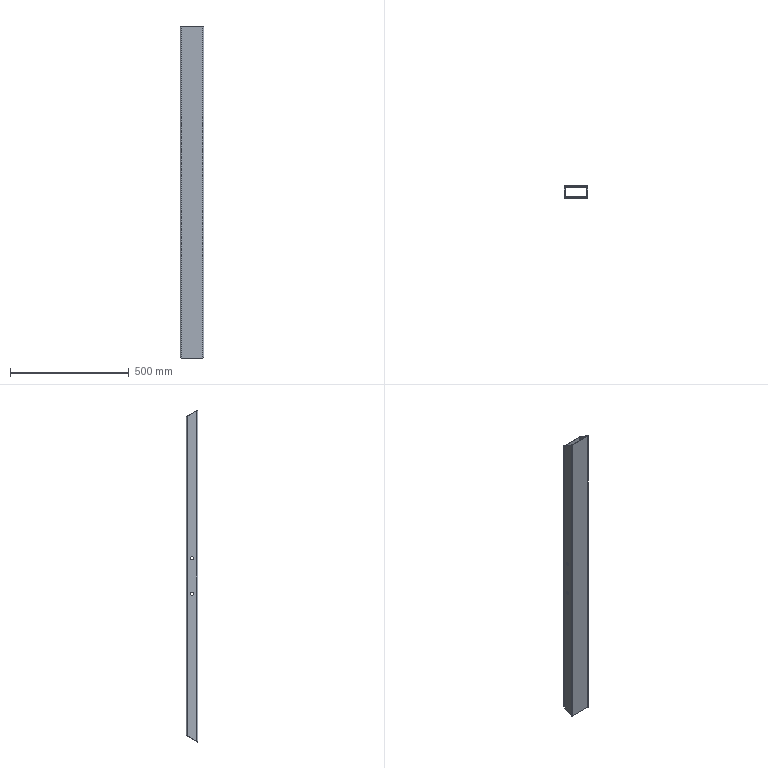Component | NX | VERTICAL_BRACKET_BASE_BEAM | 1 solid | 22 faces | volume 1555483 mm3 | cylinder 12 | plane 10 | commonest cylinder face diameters 8 x8 13 x4